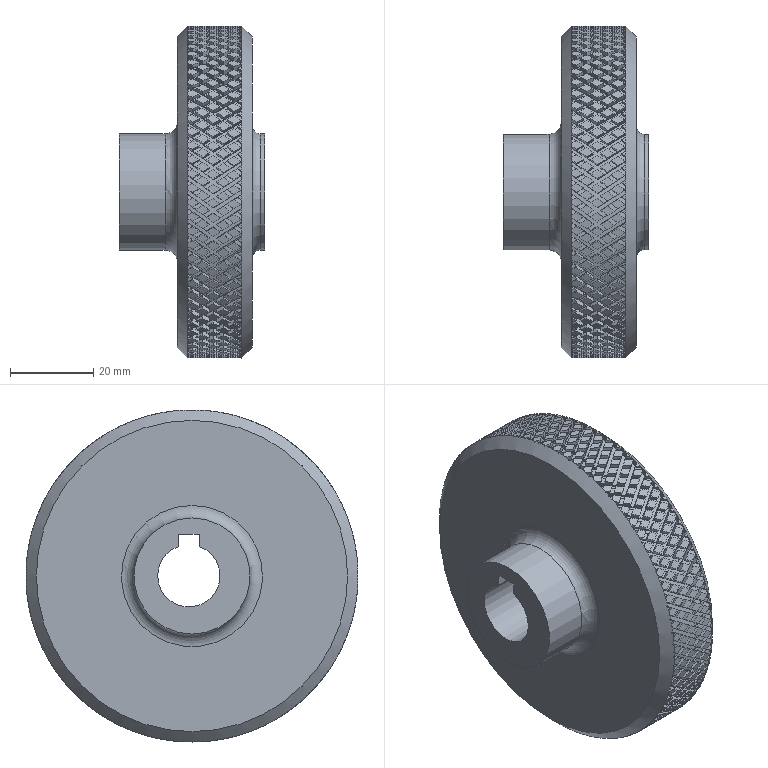Component | NX | HAND_WHEEL | 1 solid | 2246 faces | volume 90743 mm3 | plane 1735 | cylinder 507 | torus 2 | cone 2 | commonest cylinder face diameters 80 x504 28 x2 15 x1